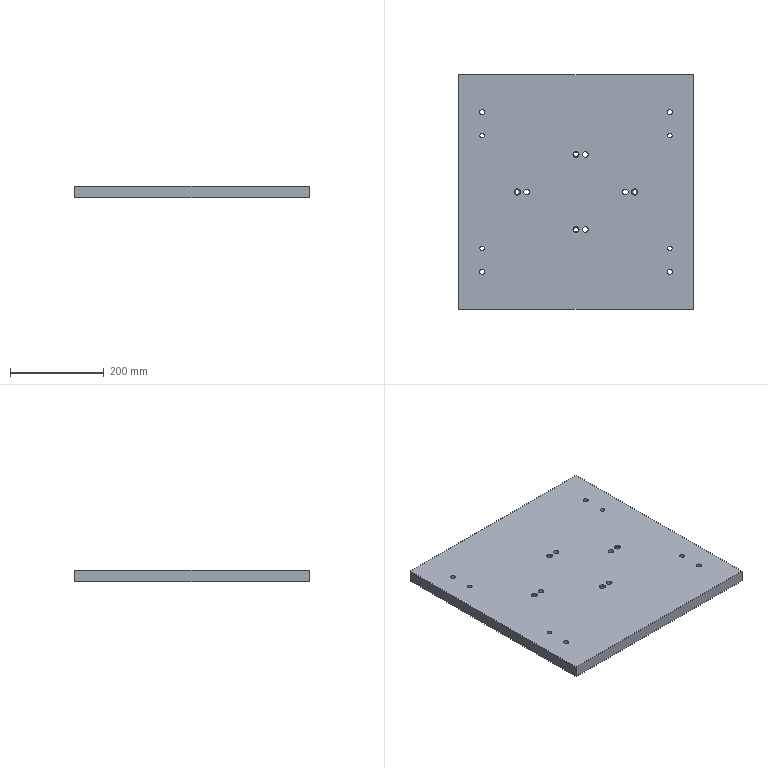Component | NX | PUNCH_FIX_PLATE | 1 solid | 30 faces | volume 6212829 mm3 | cylinder 20 | plane 10 | commonest cylinder face diameters 10 x8 13 x4 12 x4 11 x4